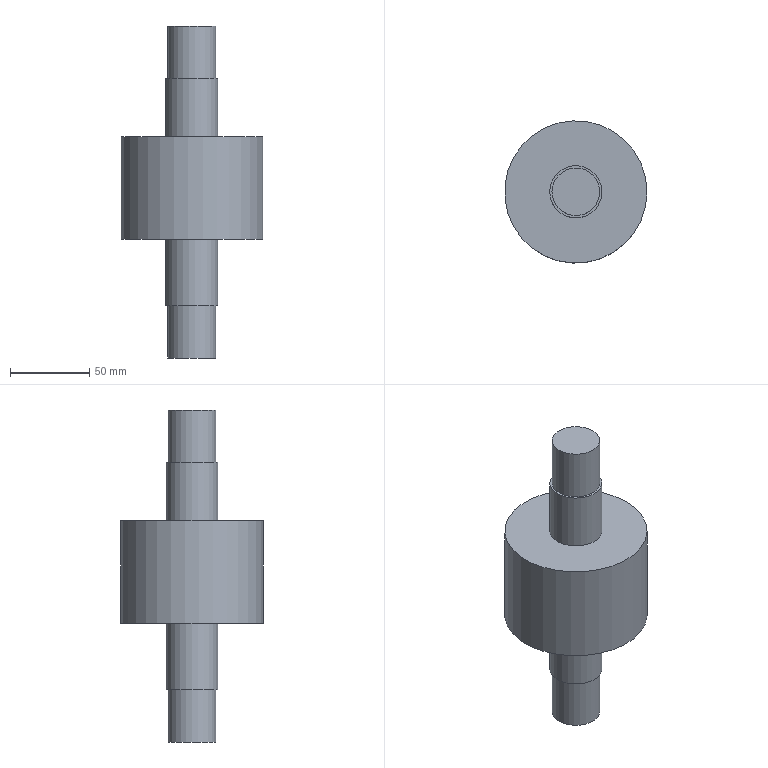Component | NX | LOCATING_PIN | 1 solid | 11 faces | box 90 x 90 x 210 mm | volume 528227 mm3 | plane 6 | cylinder 5 | commonest cylinder face diameters 33 x2 30.158 x2 90 x1
STEP:
#1=CARTESIAN_POINT('',(0.,0.,0.));
#2=DIRECTION('',(0.,0.,1.));
#3=DIRECTION('',(1.,0.,0.));
#4=AXIS2_PLACEMENT_3D('',#1,#2,#3);
#5=CARTESIAN_POINT('',(45.,0.,98.));
#6=VERTEX_POINT('',#5);
#7=CARTESIAN_POINT('',(0.,0.,98.));
#8=DIRECTION('',(0.,0.,1.));
#9=DIRECTION('',(1.,0.,0.));
#10=AXIS2_PLACEMENT_3D('',#7,#8,#9);
#11=CIRCLE('',#10,45.);
#12=CARTESIAN_POINT('',(0.,0.,98.));
#13=DIRECTION('',(0.,0.,-1.));
#14=DIRECTION('',(-1.,0.,0.));
#15=AXIS2_PLACEMENT_3D('',#12,#13,#14);
#16=CYLINDRICAL_SURFACE('',#15,45.);
#17=CARTESIAN_POINT('',(9.425,0.));
#18=DIRECTION('',(-1.,0.));
#19=VECTOR('',#18,1.);
#20=LINE('',#17,#19);
#21=(GEOMETRIC_REPRESENTATION_CONTEXT(2)PARAMETRIC_REPRESENTATION_CONTEXT()REPRESENTATION_CONTEXT('',''));
#22=DEFINITIONAL_REPRESENTATION('',(#20),#21);
#23=PCURVE('',#16,#22);
#24=CARTESIAN_POINT('',(0.,0.,98.));
#25=DIRECTION('',(0.,0.,1.));
#26=DIRECTION('',(1.,0.,0.));
#27=AXIS2_PLACEMENT_3D('',#24,#25,#26);
#28=PLANE('',#27);
#29=CARTESIAN_POINT('',(0.,0.));
#30=DIRECTION('',(1.,0.));
#31=AXIS2_PLACEMENT_2D('',#29,#30);
#32=CIRCLE('',#31,45.);
#33=(GEOMETRIC_REPRESENTATION_CONTEXT(2)PARAMETRIC_REPRESENTATION_CONTEXT()REPRESENTATION_CONTEXT('',''));
#34=DEFINITIONAL_REPRESENTATION('',(#32),#33);
#35=PCURVE('',#28,#34);
#36=SURFACE_CURVE('',#11,(#23,#35),.PCURVE_S1.);
#37=EDGE_CURVE('',#6,#6,#36,.T.);
#38=ORIENTED_EDGE('',*,*,#37,.F.);
#39=CARTESIAN_POINT('',(45.,0.,33.));
#40=VERTEX_POINT('',#39);
#41=CARTESIAN_POINT('',(45.,0.,98.));
#42=CARTESIAN_POINT('',(45.,0.,33.));
#43=B_SPLINE_CURVE_WITH_KNOTS('',1,(#41,#42),.UNSPECIFIED.,.F.,.F.,(2,2),(0.,65.),.PIECEWISE_BEZIER_KNOTS.);
#44=CARTESIAN_POINT('',(9.425,0.));
#45=DIRECTION('',(0.,1.));
#46=VECTOR('',#45,1.);
#47=LINE('',#44,#46);
#48=(GEOMETRIC_REPRESENTATION_CONTEXT(2)PARAMETRIC_REPRESENTATION_CONTEXT()REPRESENTATION_CONTEXT('',''));
#49=DEFINITIONAL_REPRESENTATION('',(#47),#48);
#50=PCURVE('',#16,#49);
#51=CARTESIAN_POINT('',(3.142,0.));
#52=DIRECTION('',(0.,1.));
#53=VECTOR('',#52,1.);
#54=LINE('',#51,#53);
#55=(GEOMETRIC_REPRESENTATION_CONTEXT(2)PARAMETRIC_REPRESENTATION_CONTEXT()REPRESENTATION_CONTEXT('',''));
#56=DEFINITIONAL_REPRESENTATION('',(#54),#55);
#57=PCURVE('',#16,#56);
#58=SEAM_CURVE('',#43,(#50,#57),.PCURVE_S1.);
#59=EDGE_CURVE('',#6,#40,#58,.T.);
#60=ORIENTED_EDGE('',*,*,#59,.T.);
#61=CARTESIAN_POINT('',(0.,0.,33.));
#62=DIRECTION('',(0.,0.,1.));
#63=DIRECTION('',(1.,0.,0.));
#64=AXIS2_PLACEMENT_3D('',#61,#62,#63);
#65=CIRCLE('',#64,45.);
#66=CARTESIAN_POINT('',(9.425,65.));
#67=DIRECTION('',(-1.,0.));
#68=VECTOR('',#67,1.);
#69=LINE('',#66,#68);
#70=(GEOMETRIC_REPRESENTATION_CONTEXT(2)PARAMETRIC_REPRESENTATION_CONTEXT()REPRESENTATION_CONTEXT('',''));
#71=DEFINITIONAL_REPRESENTATION('',(#69),#70);
#72=PCURVE('',#16,#71);
#73=CARTESIAN_POINT('',(0.,0.,33.));
#74=DIRECTION('',(0.,0.,1.));
#75=DIRECTION('',(1.,0.,0.));
#76=AXIS2_PLACEMENT_3D('',#73,#74,#75);
#77=PLANE('',#76);
#78=CARTESIAN_POINT('',(0.,0.));
#79=DIRECTION('',(1.,0.));
#80=AXIS2_PLACEMENT_2D('',#78,#79);
#81=CIRCLE('',#80,45.);
#82=(GEOMETRIC_REPRESENTATION_CONTEXT(2)PARAMETRIC_REPRESENTATION_CONTEXT()REPRESENTATION_CONTEXT('',''));
#83=DEFINITIONAL_REPRESENTATION('',(#81),#82);
#84=PCURVE('',#77,#83);
#85=SURFACE_CURVE('',#65,(#72,#84),.PCURVE_S1.);
#86=EDGE_CURVE('',#40,#40,#85,.T.);
#87=ORIENTED_EDGE('',*,*,#86,.T.);
#88=ORIENTED_EDGE('',*,*,#59,.F.);
#89=EDGE_LOOP('',(#38,#60,#87,#88));
#90=FACE_BOUND('',#89,.T.);
#91=ADVANCED_FACE('',(#90),#16,.T.);
#92=CARTESIAN_POINT('',(16.5,0.,98.));
#93=VERTEX_POINT('',#92);
#94=CARTESIAN_POINT('',(-16.5,0.,98.));
#95=VERTEX_POINT('',#94);
#96=CARTESIAN_POINT('',(0.,0.,98.));
#97=DIRECTION('',(0.,0.,1.));
#98=DIRECTION('',(1.,0.,0.));
#99=AXIS2_PLACEMENT_3D('',#96,#97,#98);
#100=CIRCLE('',#99,16.5);
#101=CARTESIAN_POINT('',(0.,0.));
#102=DIRECTION('',(1.,0.));
#103=AXIS2_PLACEMENT_2D('',#101,#102);
#104=CIRCLE('',#103,16.5);
#105=(GEOMETRIC_REPRESENTATION_CONTEXT(2)PARAMETRIC_REPRESENTATION_CONTEXT()REPRESENTATION_CONTEXT('',''));
#106=DEFINITIONAL_REPRESENTATION('',(#104),#105);
#107=PCURVE('',#28,#106);
#108=CARTESIAN_POINT('',(0.,0.,168.));
#109=DIRECTION('',(0.,0.,-1.));
#110=DIRECTION('',(-1.,0.,0.));
#111=AXIS2_PLACEMENT_3D('',#108,#109,#110);
#112=CYLINDRICAL_SURFACE('',#111,16.5);
#113=CARTESIAN_POINT('',(3.142,70.));
#114=DIRECTION('',(-1.,0.));
#115=VECTOR('',#114,1.);
#116=LINE('',#113,#115);
#117=(GEOMETRIC_REPRESENTATION_CONTEXT(2)PARAMETRIC_REPRESENTATION_CONTEXT()REPRESENTATION_CONTEXT('',''));
#118=DEFINITIONAL_REPRESENTATION('',(#116),#117);
#119=PCURVE('',#112,#118);
#120=SURFACE_CURVE('',#100,(#107,#119),.PCURVE_S1.);
#121=EDGE_CURVE('',#93,#95,#120,.T.);
#122=ORIENTED_EDGE('',*,*,#121,.F.);
#123=CARTESIAN_POINT('',(0.,0.,98.));
#124=DIRECTION('',(0.,0.,1.));
#125=DIRECTION('',(1.,0.,0.));
#126=AXIS2_PLACEMENT_3D('',#123,#124,#125);
#127=CIRCLE('',#126,16.5);
#128=CARTESIAN_POINT('',(0.,0.));
#129=DIRECTION('',(1.,0.));
#130=AXIS2_PLACEMENT_2D('',#128,#129);
#131=CIRCLE('',#130,16.5);
#132=(GEOMETRIC_REPRESENTATION_CONTEXT(2)PARAMETRIC_REPRESENTATION_CONTEXT()REPRESENTATION_CONTEXT('',''));
#133=DEFINITIONAL_REPRESENTATION('',(#131),#132);
#134=PCURVE('',#28,#133);
#135=CARTESIAN_POINT('',(9.425,70.));
#136=DIRECTION('',(-1.,0.));
#137=VECTOR('',#136,1.);
#138=LINE('',#135,#137);
#139=(GEOMETRIC_REPRESENTATION_CONTEXT(2)PARAMETRIC_REPRESENTATION_CONTEXT()REPRESENTATION_CONTEXT('',''));
#140=DEFINITIONAL_REPRESENTATION('',(#138),#139);
#141=PCURVE('',#112,#140);
#142=SURFACE_CURVE('',#127,(#134,#141),.PCURVE_S1.);
#143=EDGE_CURVE('',#95,#93,#142,.T.);
#144=ORIENTED_EDGE('',*,*,#143,.F.);
#145=EDGE_LOOP('',(#122,#144));
#146=FACE_BOUND('',#145,.T.);
#147=ORIENTED_EDGE('',*,*,#37,.T.);
#148=EDGE_LOOP('',(#147));
#149=FACE_BOUND('',#148,.T.);
#150=ADVANCED_FACE('',(#146,#149),#28,.T.);
#151=CARTESIAN_POINT('',(16.5,0.,33.));
#152=VERTEX_POINT('',#151);
#153=CARTESIAN_POINT('',(0.,0.,33.));
#154=DIRECTION('',(0.,0.,-1.));
#155=DIRECTION('',(1.,0.,0.));
#156=AXIS2_PLACEMENT_3D('',#153,#154,#155);
#157=CIRCLE('',#156,16.5);
#158=CARTESIAN_POINT('',(16.5,0.));
#159=CARTESIAN_POINT('',(16.5,-28.579));
#160=CARTESIAN_POINT('',(-8.25,-14.289));
#161=CARTESIAN_POINT('',(-33.,-0.));
#162=CARTESIAN_POINT('',(-8.25,14.289));
#163=CARTESIAN_POINT('',(16.5,28.579));
#164=CARTESIAN_POINT('',(16.5,0.));
#165=(BOUNDED_CURVE()B_SPLINE_CURVE(2,(#158,#159,#160,#161,#162,#163,#164),.UNSPECIFIED.,.T.,.F.)B_SPLINE_CURVE_WITH_KNOTS((1,2,2,2,2,1),(-2.094,0.,2.094,4.189,6.283,8.378),.UNSPECIFIED.)CURVE()GEOMETRIC_REPRESENTATION_ITEM()RATIONAL_B_SPLINE_CURVE((1.,0.5,1.,0.5,1.,0.5,1.))REPRESENTATION_ITEM(''));
#166=(GEOMETRIC_REPRESENTATION_CONTEXT(2)PARAMETRIC_REPRESENTATION_CONTEXT()REPRESENTATION_CONTEXT('',''));
#167=DEFINITIONAL_REPRESENTATION('',(#165),#166);
#168=PCURVE('',#77,#167);
#169=CARTESIAN_POINT('',(0.,0.,-42.));
#170=DIRECTION('',(0.,0.,1.));
#171=DIRECTION('',(1.,0.,0.));
#172=AXIS2_PLACEMENT_3D('',#169,#170,#171);
#173=CYLINDRICAL_SURFACE('',#172,16.5);
#174=CARTESIAN_POINT('',(6.283,75.));
#175=DIRECTION('',(-1.,0.));
#176=VECTOR('',#175,1.);
#177=LINE('',#174,#176);
#178=(GEOMETRIC_REPRESENTATION_CONTEXT(2)PARAMETRIC_REPRESENTATION_CONTEXT()REPRESENTATION_CONTEXT('',''));
#179=DEFINITIONAL_REPRESENTATION('',(#177),#178);
#180=PCURVE('',#173,#179);
#181=SURFACE_CURVE('',#157,(#168,#180),.PCURVE_S1.);
#182=EDGE_CURVE('',#152,#152,#181,.T.);
#183=ORIENTED_EDGE('',*,*,#182,.F.);
#184=EDGE_LOOP('',(#183));
#185=FACE_BOUND('',#184,.T.);
#186=ORIENTED_EDGE('',*,*,#86,.F.);
#187=EDGE_LOOP('',(#186));
#188=FACE_BOUND('',#187,.T.);
#189=ADVANCED_FACE('',(#185,#188),#77,.F.);
#190=CARTESIAN_POINT('',(-16.5,0.,135.));
#191=VERTEX_POINT('',#190);
#192=CARTESIAN_POINT('',(0.,0.,135.));
#193=DIRECTION('',(0.,0.,-1.));
#194=DIRECTION('',(-1.,0.,0.));
#195=AXIS2_PLACEMENT_3D('',#192,#193,#194);
#196=CIRCLE('',#195,16.5);
#197=CARTESIAN_POINT('',(0.,33.));
#198=DIRECTION('',(1.,0.));
#199=VECTOR('',#198,1.);
#200=LINE('',#197,#199);
#201=(GEOMETRIC_REPRESENTATION_CONTEXT(2)PARAMETRIC_REPRESENTATION_CONTEXT()REPRESENTATION_CONTEXT('',''));
#202=DEFINITIONAL_REPRESENTATION('',(#200),#201);
#203=PCURVE('',#112,#202);
#204=CARTESIAN_POINT('',(0.,0.,135.));
#205=DIRECTION('',(0.,0.,-1.));
#206=DIRECTION('',(-1.,0.,0.));
#207=AXIS2_PLACEMENT_3D('',#204,#205,#206);
#208=PLANE('',#207);
#209=CARTESIAN_POINT('',(0.,0.));
#210=DIRECTION('',(1.,0.));
#211=AXIS2_PLACEMENT_2D('',#209,#210);
#212=CIRCLE('',#211,16.5);
#213=(GEOMETRIC_REPRESENTATION_CONTEXT(2)PARAMETRIC_REPRESENTATION_CONTEXT()REPRESENTATION_CONTEXT('',''));
#214=DEFINITIONAL_REPRESENTATION('',(#212),#213);
#215=PCURVE('',#208,#214);
#216=SURFACE_CURVE('',#196,(#203,#215),.PCURVE_S1.);
#217=EDGE_CURVE('',#191,#191,#216,.T.);
#218=ORIENTED_EDGE('',*,*,#217,.T.);
#219=CARTESIAN_POINT('',(-16.5,0.,135.));
#220=CARTESIAN_POINT('',(-16.5,0.,98.));
#221=B_SPLINE_CURVE_WITH_KNOTS('',1,(#219,#220),.UNSPECIFIED.,.F.,.F.,(2,2),(33.,70.),.PIECEWISE_BEZIER_KNOTS.);
#222=CARTESIAN_POINT('',(6.283,0.));
#223=DIRECTION('',(0.,1.));
#224=VECTOR('',#223,1.);
#225=LINE('',#222,#224);
#226=(GEOMETRIC_REPRESENTATION_CONTEXT(2)PARAMETRIC_REPRESENTATION_CONTEXT()REPRESENTATION_CONTEXT('',''));
#227=DEFINITIONAL_REPRESENTATION('',(#225),#226);
#228=PCURVE('',#112,#227);
#229=CARTESIAN_POINT('',(0.,0.));
#230=DIRECTION('',(0.,1.));
#231=VECTOR('',#230,1.);
#232=LINE('',#229,#231);
#233=(GEOMETRIC_REPRESENTATION_CONTEXT(2)PARAMETRIC_REPRESENTATION_CONTEXT()REPRESENTATION_CONTEXT('',''));
#234=DEFINITIONAL_REPRESENTATION('',(#232),#233);
#235=PCURVE('',#112,#234);
#236=SEAM_CURVE('',#221,(#228,#235),.PCURVE_S1.);
#237=EDGE_CURVE('',#191,#95,#236,.T.);
#238=ORIENTED_EDGE('',*,*,#237,.T.);
#239=ORIENTED_EDGE('',*,*,#143,.T.);
#240=ORIENTED_EDGE('',*,*,#121,.T.);
#241=ORIENTED_EDGE('',*,*,#237,.F.);
#242=EDGE_LOOP('',(#218,#238,#239,#240,#241));
#243=FACE_BOUND('',#242,.T.);
#244=ADVANCED_FACE('',(#243),#112,.T.);
#245=CARTESIAN_POINT('',(16.5,0.,-9.));
#246=VERTEX_POINT('',#245);
#247=CARTESIAN_POINT('',(0.,0.,-9.));
#248=DIRECTION('',(0.,0.,1.));
#249=DIRECTION('',(1.,0.,0.));
#250=AXIS2_PLACEMENT_3D('',#247,#248,#249);
#251=CIRCLE('',#250,16.5);
#252=CARTESIAN_POINT('',(0.,33.));
#253=DIRECTION('',(1.,0.));
#254=VECTOR('',#253,1.);
#255=LINE('',#252,#254);
#256=(GEOMETRIC_REPRESENTATION_CONTEXT(2)PARAMETRIC_REPRESENTATION_CONTEXT()REPRESENTATION_CONTEXT('',''));
#257=DEFINITIONAL_REPRESENTATION('',(#255),#256);
#258=PCURVE('',#173,#257);
#259=CARTESIAN_POINT('',(0.,0.,-9.));
#260=DIRECTION('',(0.,0.,1.));
#261=DIRECTION('',(1.,0.,0.));
#262=AXIS2_PLACEMENT_3D('',#259,#260,#261);
#263=PLANE('',#262);
#264=CARTESIAN_POINT('',(0.,0.));
#265=DIRECTION('',(1.,0.));
#266=AXIS2_PLACEMENT_2D('',#264,#265);
#267=CIRCLE('',#266,16.5);
#268=(GEOMETRIC_REPRESENTATION_CONTEXT(2)PARAMETRIC_REPRESENTATION_CONTEXT()REPRESENTATION_CONTEXT('',''));
#269=DEFINITIONAL_REPRESENTATION('',(#267),#268);
#270=PCURVE('',#263,#269);
#271=SURFACE_CURVE('',#251,(#258,#270),.PCURVE_S1.);
#272=EDGE_CURVE('',#246,#246,#271,.T.);
#273=ORIENTED_EDGE('',*,*,#272,.T.);
#274=CARTESIAN_POINT('',(16.5,0.,-9.));
#275=CARTESIAN_POINT('',(16.5,0.,33.));
#276=B_SPLINE_CURVE_WITH_KNOTS('',1,(#274,#275),.UNSPECIFIED.,.F.,.F.,(2,2),(33.,75.),.PIECEWISE_BEZIER_KNOTS.);
#277=CARTESIAN_POINT('',(6.283,0.));
#278=DIRECTION('',(0.,1.));
#279=VECTOR('',#278,1.);
#280=LINE('',#277,#279);
#281=(GEOMETRIC_REPRESENTATION_CONTEXT(2)PARAMETRIC_REPRESENTATION_CONTEXT()REPRESENTATION_CONTEXT('',''));
#282=DEFINITIONAL_REPRESENTATION('',(#280),#281);
#283=PCURVE('',#173,#282);
#284=CARTESIAN_POINT('',(0.,0.));
#285=DIRECTION('',(0.,1.));
#286=VECTOR('',#285,1.);
#287=LINE('',#284,#286);
#288=(GEOMETRIC_REPRESENTATION_CONTEXT(2)PARAMETRIC_REPRESENTATION_CONTEXT()REPRESENTATION_CONTEXT('',''));
#289=DEFINITIONAL_REPRESENTATION('',(#287),#288);
#290=PCURVE('',#173,#289);
#291=SEAM_CURVE('',#276,(#283,#290),.PCURVE_S1.);
#292=EDGE_CURVE('',#246,#152,#291,.T.);
#293=ORIENTED_EDGE('',*,*,#292,.T.);
#294=ORIENTED_EDGE('',*,*,#182,.T.);
#295=ORIENTED_EDGE('',*,*,#292,.F.);
#296=EDGE_LOOP('',(#273,#293,#294,#295));
#297=FACE_BOUND('',#296,.T.);
#298=ADVANCED_FACE('',(#297),#173,.T.);
#299=CARTESIAN_POINT('',(15.079,0.,-9.));
#300=VERTEX_POINT('',#299);
#301=CARTESIAN_POINT('',(0.,0.,-9.));
#302=DIRECTION('',(0.,0.,-1.));
#303=DIRECTION('',(1.,0.,0.));
#304=AXIS2_PLACEMENT_3D('',#301,#302,#303);
#305=CIRCLE('',#304,15.079);
#306=CARTESIAN_POINT('',(15.079,0.));
#307=CARTESIAN_POINT('',(15.079,-26.118));
#308=CARTESIAN_POINT('',(-7.54,-13.059));
#309=CARTESIAN_POINT('',(-30.158,-0.));
#310=CARTESIAN_POINT('',(-7.54,13.059));
#311=CARTESIAN_POINT('',(15.079,26.118));
#312=CARTESIAN_POINT('',(15.079,0.));
#313=(BOUNDED_CURVE()B_SPLINE_CURVE(2,(#306,#307,#308,#309,#310,#311,#312),.UNSPECIFIED.,.T.,.F.)B_SPLINE_CURVE_WITH_KNOTS((1,2,2,2,2,1),(-2.094,0.,2.094,4.189,6.283,8.378),.UNSPECIFIED.)CURVE()GEOMETRIC_REPRESENTATION_ITEM()RATIONAL_B_SPLINE_CURVE((1.,0.5,1.,0.5,1.,0.5,1.))REPRESENTATION_ITEM(''));
#314=(GEOMETRIC_REPRESENTATION_CONTEXT(2)PARAMETRIC_REPRESENTATION_CONTEXT()REPRESENTATION_CONTEXT('',''));
#315=DEFINITIONAL_REPRESENTATION('',(#313),#314);
#316=PCURVE('',#263,#315);
#317=CARTESIAN_POINT('',(0.,0.,-44.));
#318=DIRECTION('',(0.,0.,1.));
#319=DIRECTION('',(1.,0.,0.));
#320=AXIS2_PLACEMENT_3D('',#317,#318,#319);
#321=CYLINDRICAL_SURFACE('',#320,15.079);
#322=CARTESIAN_POINT('',(6.283,35.));
#323=DIRECTION('',(-1.,0.));
#324=VECTOR('',#323,1.);
#325=LINE('',#322,#324);
#326=(GEOMETRIC_REPRESENTATION_CONTEXT(2)PARAMETRIC_REPRESENTATION_CONTEXT()REPRESENTATION_CONTEXT('',''));
#327=DEFINITIONAL_REPRESENTATION('',(#325),#326);
#328=PCURVE('',#321,#327);
#329=SURFACE_CURVE('',#305,(#316,#328),.PCURVE_S1.);
#330=EDGE_CURVE('',#300,#300,#329,.T.);
#331=ORIENTED_EDGE('',*,*,#330,.F.);
#332=EDGE_LOOP('',(#331));
#333=FACE_BOUND('',#332,.T.);
#334=ORIENTED_EDGE('',*,*,#272,.F.);
#335=EDGE_LOOP('',(#334));
#336=FACE_BOUND('',#335,.T.);
#337=ADVANCED_FACE('',(#333,#336),#263,.F.);
#338=CARTESIAN_POINT('',(15.079,-0.,-42.));
#339=VERTEX_POINT('',#338);
#340=CARTESIAN_POINT('',(-15.079,0.,-42.));
#341=VERTEX_POINT('',#340);
#342=CARTESIAN_POINT('',(0.,0.,-42.));
#343=DIRECTION('',(0.,0.,-1.));
#344=DIRECTION('',(-1.,0.,0.));
#345=AXIS2_PLACEMENT_3D('',#342,#343,#344);
#346=CIRCLE('',#345,15.079);
#347=CARTESIAN_POINT('',(9.425,2.));
#348=DIRECTION('',(-1.,0.));
#349=VECTOR('',#348,1.);
#350=LINE('',#347,#349);
#351=(GEOMETRIC_REPRESENTATION_CONTEXT(2)PARAMETRIC_REPRESENTATION_CONTEXT()REPRESENTATION_CONTEXT('',''));
#352=DEFINITIONAL_REPRESENTATION('',(#350),#351);
#353=PCURVE('',#321,#352);
#354=CARTESIAN_POINT('',(0.,0.,-42.));
#355=DIRECTION('',(0.,0.,-1.));
#356=DIRECTION('',(-1.,0.,0.));
#357=AXIS2_PLACEMENT_3D('',#354,#355,#356);
#358=PLANE('',#357);
#359=CARTESIAN_POINT('',(0.,0.));
#360=DIRECTION('',(1.,0.));
#361=AXIS2_PLACEMENT_2D('',#359,#360);
#362=CIRCLE('',#361,15.079);
#363=(GEOMETRIC_REPRESENTATION_CONTEXT(2)PARAMETRIC_REPRESENTATION_CONTEXT()REPRESENTATION_CONTEXT('',''));
#364=DEFINITIONAL_REPRESENTATION('',(#362),#363);
#365=PCURVE('',#358,#364);
#366=SURFACE_CURVE('',#346,(#353,#365),.PCURVE_S1.);
#367=EDGE_CURVE('',#339,#341,#366,.T.);
#368=ORIENTED_EDGE('',*,*,#367,.F.);
#369=CARTESIAN_POINT('',(15.079,0.,-42.));
#370=CARTESIAN_POINT('',(15.079,0.,-9.));
#371=B_SPLINE_CURVE_WITH_KNOTS('',1,(#369,#370),.UNSPECIFIED.,.F.,.F.,(2,2),(2.,35.),.PIECEWISE_BEZIER_KNOTS.);
#372=CARTESIAN_POINT('',(6.283,0.));
#373=DIRECTION('',(0.,1.));
#374=VECTOR('',#373,1.);
#375=LINE('',#372,#374);
#376=(GEOMETRIC_REPRESENTATION_CONTEXT(2)PARAMETRIC_REPRESENTATION_CONTEXT()REPRESENTATION_CONTEXT('',''));
#377=DEFINITIONAL_REPRESENTATION('',(#375),#376);
#378=PCURVE('',#321,#377);
#379=CARTESIAN_POINT('',(0.,0.));
#380=DIRECTION('',(0.,1.));
#381=VECTOR('',#380,1.);
#382=LINE('',#379,#381);
#383=(GEOMETRIC_REPRESENTATION_CONTEXT(2)PARAMETRIC_REPRESENTATION_CONTEXT()REPRESENTATION_CONTEXT('',''));
#384=DEFINITIONAL_REPRESENTATION('',(#382),#383);
#385=PCURVE('',#321,#384);
#386=SEAM_CURVE('',#371,(#378,#385),.PCURVE_S1.);
#387=EDGE_CURVE('',#339,#300,#386,.T.);
#388=ORIENTED_EDGE('',*,*,#387,.T.);
#389=ORIENTED_EDGE('',*,*,#330,.T.);
#390=ORIENTED_EDGE('',*,*,#387,.F.);
#391=CARTESIAN_POINT('',(0.,0.,-42.));
#392=DIRECTION('',(0.,0.,-1.));
#393=DIRECTION('',(-1.,0.,0.));
#394=AXIS2_PLACEMENT_3D('',#391,#392,#393);
#395=CIRCLE('',#394,15.079);
#396=CARTESIAN_POINT('',(3.142,2.));
#397=DIRECTION('',(-1.,0.));
#398=VECTOR('',#397,1.);
#399=LINE('',#396,#398);
#400=(GEOMETRIC_REPRESENTATION_CONTEXT(2)PARAMETRIC_REPRESENTATION_CONTEXT()REPRESENTATION_CONTEXT('',''));
#401=DEFINITIONAL_REPRESENTATION('',(#399),#400);
#402=PCURVE('',#321,#401);
#403=CARTESIAN_POINT('',(0.,0.));
#404=DIRECTION('',(1.,0.));
#405=AXIS2_PLACEMENT_2D('',#403,#404);
#406=CIRCLE('',#405,15.079);
#407=(GEOMETRIC_REPRESENTATION_CONTEXT(2)PARAMETRIC_REPRESENTATION_CONTEXT()REPRESENTATION_CONTEXT('',''));
#408=DEFINITIONAL_REPRESENTATION('',(#406),#407);
#409=PCURVE('',#358,#408);
#410=SURFACE_CURVE('',#395,(#402,#409),.PCURVE_S1.);
#411=EDGE_CURVE('',#341,#339,#410,.T.);
#412=ORIENTED_EDGE('',*,*,#411,.F.);
#413=EDGE_LOOP('',(#368,#388,#389,#390,#412));
#414=FACE_BOUND('',#413,.T.);
#415=ADVANCED_FACE('',(#414),#321,.T.);
#416=ORIENTED_EDGE('',*,*,#411,.T.);
#417=ORIENTED_EDGE('',*,*,#367,.T.);
#418=EDGE_LOOP('',(#416,#417));
#419=FACE_BOUND('',#418,.T.);
#420=ADVANCED_FACE('',(#419),#358,.T.);
#421=CARTESIAN_POINT('',(-15.079,0.,135.));
#422=VERTEX_POINT('',#421);
#423=CARTESIAN_POINT('',(15.079,-0.,135.));
#424=VERTEX_POINT('',#423);
#425=CARTESIAN_POINT('',(0.,0.,135.));
#426=DIRECTION('',(0.,0.,1.));
#427=DIRECTION('',(-1.,0.,0.));
#428=AXIS2_PLACEMENT_3D('',#425,#426,#427);
#429=CIRCLE('',#428,15.079);
#430=CARTESIAN_POINT('',(15.079,0.));
#431=CARTESIAN_POINT('',(15.079,-26.118));
#432=CARTESIAN_POINT('',(-7.54,-13.059));
#433=CARTESIAN_POINT('',(-30.158,-0.));
#434=CARTESIAN_POINT('',(-7.54,13.059));
#435=CARTESIAN_POINT('',(15.079,26.118));
#436=CARTESIAN_POINT('',(15.079,0.));
#437=(BOUNDED_CURVE()B_SPLINE_CURVE(2,(#430,#431,#432,#433,#434,#435,#436),.UNSPECIFIED.,.T.,.F.)B_SPLINE_CURVE_WITH_KNOTS((1,2,2,2,2,1),(-2.094,0.,2.094,4.189,6.283,8.378),.UNSPECIFIED.)CURVE()GEOMETRIC_REPRESENTATION_ITEM()RATIONAL_B_SPLINE_CURVE((1.,0.5,1.,0.5,1.,0.5,1.))REPRESENTATION_ITEM(''));
#438=(GEOMETRIC_REPRESENTATION_CONTEXT(2)PARAMETRIC_REPRESENTATION_CONTEXT()REPRESENTATION_CONTEXT('',''));
#439=DEFINITIONAL_REPRESENTATION('',(#437),#438);
#440=PCURVE('',#208,#439);
#441=CARTESIAN_POINT('',(0.,0.,134.));
#442=DIRECTION('',(0.,0.,1.));
#443=DIRECTION('',(1.,0.,0.));
#444=AXIS2_PLACEMENT_3D('',#441,#442,#443);
#445=CYLINDRICAL_SURFACE('',#444,15.079);
#446=CARTESIAN_POINT('',(3.142,1.));
#447=DIRECTION('',(1.,0.));
#448=VECTOR('',#447,1.);
#449=LINE('',#446,#448);
#450=(GEOMETRIC_REPRESENTATION_CONTEXT(2)PARAMETRIC_REPRESENTATION_CONTEXT()REPRESENTATION_CONTEXT('',''));
#451=DEFINITIONAL_REPRESENTATION('',(#449),#450);
#452=PCURVE('',#445,#451);
#453=SURFACE_CURVE('',#429,(#440,#452),.PCURVE_S1.);
#454=EDGE_CURVE('',#422,#424,#453,.T.);
#455=ORIENTED_EDGE('',*,*,#454,.F.);
#456=CARTESIAN_POINT('',(0.,0.,135.));
#457=DIRECTION('',(0.,0.,1.));
#458=DIRECTION('',(-1.,0.,0.));
#459=AXIS2_PLACEMENT_3D('',#456,#457,#458);
#460=CIRCLE('',#459,15.079);
#461=CARTESIAN_POINT('',(15.079,0.));
#462=CARTESIAN_POINT('',(15.079,-26.118));
#463=CARTESIAN_POINT('',(-7.54,-13.059));
#464=CARTESIAN_POINT('',(-30.158,-0.));
#465=CARTESIAN_POINT('',(-7.54,13.059));
#466=CARTESIAN_POINT('',(15.079,26.118));
#467=CARTESIAN_POINT('',(15.079,0.));
#468=(BOUNDED_CURVE()B_SPLINE_CURVE(2,(#461,#462,#463,#464,#465,#466,#467),.UNSPECIFIED.,.T.,.F.)B_SPLINE_CURVE_WITH_KNOTS((1,2,2,2,2,1),(-2.094,0.,2.094,4.189,6.283,8.378),.UNSPECIFIED.)CURVE()GEOMETRIC_REPRESENTATION_ITEM()RATIONAL_B_SPLINE_CURVE((1.,0.5,1.,0.5,1.,0.5,1.))REPRESENTATION_ITEM(''));
#469=(GEOMETRIC_REPRESENTATION_CONTEXT(2)PARAMETRIC_REPRESENTATION_CONTEXT()REPRESENTATION_CONTEXT('',''));
#470=DEFINITIONAL_REPRESENTATION('',(#468),#469);
#471=PCURVE('',#208,#470);
#472=CARTESIAN_POINT('',(-3.142,1.));
#473=DIRECTION('',(1.,0.));
#474=VECTOR('',#473,1.);
#475=LINE('',#472,#474);
#476=(GEOMETRIC_REPRESENTATION_CONTEXT(2)PARAMETRIC_REPRESENTATION_CONTEXT()REPRESENTATION_CONTEXT('',''));
#477=DEFINITIONAL_REPRESENTATION('',(#475),#476);
#478=PCURVE('',#445,#477);
#479=SURFACE_CURVE('',#460,(#471,#478),.PCURVE_S1.);
#480=EDGE_CURVE('',#424,#422,#479,.T.);
#481=ORIENTED_EDGE('',*,*,#480,.F.);
#482=EDGE_LOOP('',(#455,#481));
#483=FACE_BOUND('',#482,.T.);
#484=ORIENTED_EDGE('',*,*,#217,.F.);
#485=EDGE_LOOP('',(#484));
#486=FACE_BOUND('',#485,.T.);
#487=ADVANCED_FACE('',(#483,#486),#208,.F.);
#488=CARTESIAN_POINT('',(15.079,0.,168.));
#489=VERTEX_POINT('',#488);
#490=CARTESIAN_POINT('',(0.,0.,168.));
#491=DIRECTION('',(0.,0.,1.));
#492=DIRECTION('',(1.,0.,0.));
#493=AXIS2_PLACEMENT_3D('',#490,#491,#492);
#494=CIRCLE('',#493,15.079);
#495=CARTESIAN_POINT('',(0.,34.));
#496=DIRECTION('',(1.,0.));
#497=VECTOR('',#496,1.);
#498=LINE('',#495,#497);
#499=(GEOMETRIC_REPRESENTATION_CONTEXT(2)PARAMETRIC_REPRESENTATION_CONTEXT()REPRESENTATION_CONTEXT('',''));
#500=DEFINITIONAL_REPRESENTATION('',(#498),#499);
#501=PCURVE('',#445,#500);
#502=CARTESIAN_POINT('',(0.,0.,168.));
#503=DIRECTION('',(0.,0.,1.));
#504=DIRECTION('',(1.,0.,0.));
#505=AXIS2_PLACEMENT_3D('',#502,#503,#504);
#506=PLANE('',#505);
#507=CARTESIAN_POINT('',(0.,0.));
#508=DIRECTION('',(1.,0.));
#509=AXIS2_PLACEMENT_2D('',#507,#508);
#510=CIRCLE('',#509,15.079);
#511=(GEOMETRIC_REPRESENTATION_CONTEXT(2)PARAMETRIC_REPRESENTATION_CONTEXT()REPRESENTATION_CONTEXT('',''));
#512=DEFINITIONAL_REPRESENTATION('',(#510),#511);
#513=PCURVE('',#506,#512);
#514=SURFACE_CURVE('',#494,(#501,#513),.PCURVE_S1.);
#515=EDGE_CURVE('',#489,#489,#514,.T.);
#516=ORIENTED_EDGE('',*,*,#515,.F.);
#517=CARTESIAN_POINT('',(15.079,-0.,135.));
#518=CARTESIAN_POINT('',(15.079,-0.,168.));
#519=B_SPLINE_CURVE_WITH_KNOTS('',1,(#517,#518),.UNSPECIFIED.,.F.,.F.,(2,2),(1.,34.),.PIECEWISE_BEZIER_KNOTS.);
#520=CARTESIAN_POINT('',(0.,0.));
#521=DIRECTION('',(0.,1.));
#522=VECTOR('',#521,1.);
#523=LINE('',#520,#522);
#524=(GEOMETRIC_REPRESENTATION_CONTEXT(2)PARAMETRIC_REPRESENTATION_CONTEXT()REPRESENTATION_CONTEXT('',''));
#525=DEFINITIONAL_REPRESENTATION('',(#523),#524);
#526=PCURVE('',#445,#525);
#527=CARTESIAN_POINT('',(6.283,0.));
#528=DIRECTION('',(0.,1.));
#529=VECTOR('',#528,1.);
#530=LINE('',#527,#529);
#531=(GEOMETRIC_REPRESENTATION_CONTEXT(2)PARAMETRIC_REPRESENTATION_CONTEXT()REPRESENTATION_CONTEXT('',''));
#532=DEFINITIONAL_REPRESENTATION('',(#530),#531);
#533=PCURVE('',#445,#532);
#534=SEAM_CURVE('',#519,(#526,#533),.PCURVE_S1.);
#535=EDGE_CURVE('',#424,#489,#534,.T.);
#536=ORIENTED_EDGE('',*,*,#535,.F.);
#537=ORIENTED_EDGE('',*,*,#480,.T.);
#538=ORIENTED_EDGE('',*,*,#454,.T.);
#539=ORIENTED_EDGE('',*,*,#535,.T.);
#540=EDGE_LOOP('',(#516,#536,#537,#538,#539));
#541=FACE_BOUND('',#540,.T.);
#542=ADVANCED_FACE('',(#541),#445,.T.);
#543=ORIENTED_EDGE('',*,*,#515,.T.);
#544=EDGE_LOOP('',(#543));
#545=FACE_BOUND('',#544,.T.);
#546=ADVANCED_FACE('',(#545),#506,.T.);
#547=CLOSED_SHELL('',(#91,#150,#189,#244,#298,#337,#415,#420,#487,#542,#546));
#548=MANIFOLD_SOLID_BREP('',#547);
#549=(LENGTH_UNIT()NAMED_UNIT(*)SI_UNIT(.MILLI.,.METRE.));
#550=UNCERTAINTY_MEASURE_WITH_UNIT(LENGTH_MEASURE(0.000005),#549,'','');
#551=(NAMED_UNIT(*)PLANE_ANGLE_UNIT()SI_UNIT($,.RADIAN.));
#552=(NAMED_UNIT(*)SI_UNIT($,.STERADIAN.)SOLID_ANGLE_UNIT());
#553=(GEOMETRIC_REPRESENTATION_CONTEXT(3)GLOBAL_UNCERTAINTY_ASSIGNED_CONTEXT((#550))GLOBAL_UNIT_ASSIGNED_CONTEXT((#549,#551,#552))REPRESENTATION_CONTEXT('',''));
#554=ADVANCED_BREP_SHAPE_REPRESENTATION('',(#4,#548),#553);